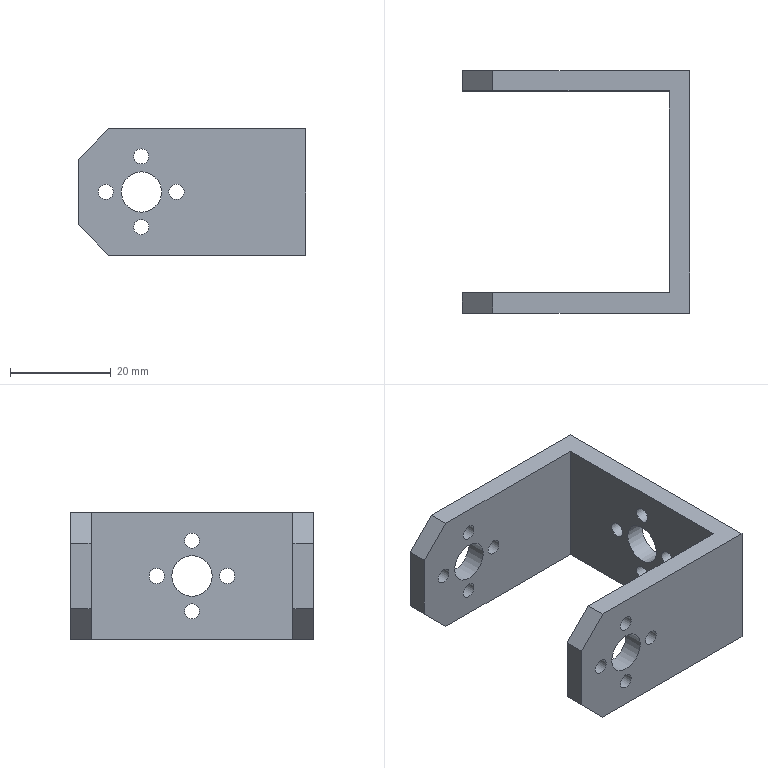Component | NX | U_SHAPE_10 | 1 solid | 29 faces | volume 11770 mm3 | cylinder 15 | plane 14 | commonest cylinder face diameters 3 x12 8 x3